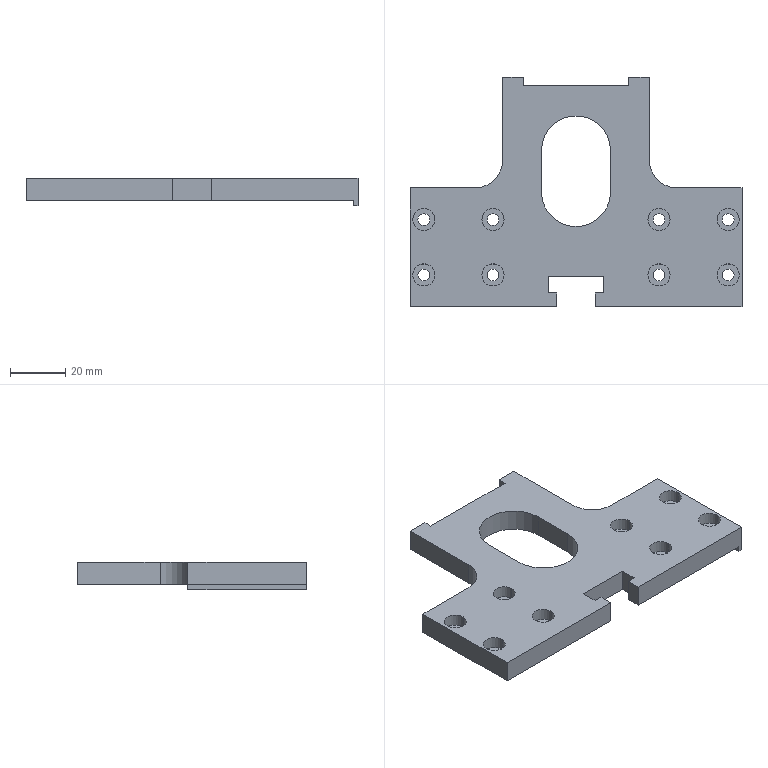Component | SolidWorks | HandlingMechanism-2_A069-1 | 1 solid | 78 faces | box 120 x 83 x 10 mm | volume 46963 mm3 | cylinder 40 | plane 34 | cone 4 | commonest cylinder face diameters 8 x16 4.3 x16 3.3 x4 25 x2 20 x2
build123d program:
from build123d import *

# Parameters (mm, degrees)
SKETCH1_W                                       = 120
SKETCH1_H                                       = 83
BOSS_EXTRUDE1_DEPTH                             = 10
SKETCH6_W                                       = 14
SKETCH6_H                                       = 5
CUT_EXTRUDE2_DEPTH                              = 15
SKETCH7_W                                       = 20
SKETCH7_H                                       = 6
CUT_EXTRUDE3_DEPTH                              = 15
SKETCH8_W                                       = 118.5
SKETCH8_H                                       = 83
CUT_EXTRUDE4_DEPTH                              = 2
SKETCH11_W                                      = 33.5
SKETCH11_H                                      = 40
CUT_EXTRUDE7_DEPTH                              = 20
SKETCH16_W                                      = 38
SKETCH16_H                                      = 3
CUT_EXTRUDE9_DEPTH                              = 20
M4_HEX_SOCKET_HEAD_CAP_SCREW_CBORE1_D           = 4.3
M4_HEX_SOCKET_HEAD_CAP_SCREW_CBORE1_CBORE_D     = 8
M4_HEX_SOCKET_HEAD_CAP_SCREW_CBORE1_CBORE_DEPTH = 4.4
CUT_EXTRUDE10_DEPTH                             = 74.636
M4_TAPPED_HOLE1_D                               = 3.3
M4_TAPPED_HOLE1_DEPTH                           = 11.5
M4_TAPPED_HOLE1_TIP                             = 0.9914
FILLET1_R                                       = 10


with BuildPart() as part:
    # Sketch1 → Boss-Extrude1 (new body)
    with BuildSketch(Plane.XY):
        Rectangle(SKETCH1_W, SKETCH1_H)
    extrude(amount=BOSS_EXTRUDE1_DEPTH)

    # Sketch6 → Cut-Extrude2 (cut)
    with BuildSketch(Plane.XY.offset(10)):
        with Locations((0, 39)):
            Rectangle(SKETCH6_W, SKETCH6_H)
    extrude(amount=-CUT_EXTRUDE2_DEPTH, mode=Mode.SUBTRACT)

    # Sketch7 → Cut-Extrude3 (cut)
    with BuildSketch(Plane.XY.offset(10)):
        with Locations((0, 33.5)):
            Rectangle(SKETCH7_W, SKETCH7_H)
    extrude(amount=-CUT_EXTRUDE3_DEPTH, mode=Mode.SUBTRACT)

    # Sketch8 → Cut-Extrude4 (cut)
    with BuildSketch(Plane(origin=(0, 0, 0), x_dir=(-1, 0, 0), z_dir=(0, 0, -1))):
        with Locations((-0.75, 0)):
            Rectangle(SKETCH8_W, SKETCH8_H)
    extrude(amount=-CUT_EXTRUDE4_DEPTH, mode=Mode.SUBTRACT)

    # Sketch11 → Cut-Extrude7 (cut)
    with BuildSketch(Plane.XY.offset(10)):
        with Locations((-43.25, -21.5)):
            Rectangle(SKETCH11_W, SKETCH11_H)
        with Locations((43.25, -21.5)):
            Rectangle(SKETCH11_W, SKETCH11_H)
    extrude(amount=-CUT_EXTRUDE7_DEPTH, mode=Mode.SUBTRACT)

    # Sketch16 → Cut-Extrude9 (cut)
    with BuildSketch(Plane(origin=(0, 0, 0), x_dir=(-1, 0, 0), z_dir=(0, 0, -1))):
        with Locations((0, -40)):
            Rectangle(SKETCH16_W, SKETCH16_H)
    extrude(amount=-CUT_EXTRUDE9_DEPTH, mode=Mode.SUBTRACT)

    # M4 Hex Socket Head Cap Screw CBORE1 (through all)
    with Locations(Plane.XY.offset(10)):
        with Locations((-55, 10), (-55, 30), (-30, 30), (-30, 10), (55, 30), (30, 30), (30, 10), (55, 10)):
            CounterBoreHole(M4_HEX_SOCKET_HEAD_CAP_SCREW_CBORE1_D / 2, M4_HEX_SOCKET_HEAD_CAP_SCREW_CBORE1_CBORE_D / 2, M4_HEX_SOCKET_HEAD_CAP_SCREW_CBORE1_CBORE_DEPTH)

    # Sketch19 → Cut-Extrude10 (cut, through all)
    with BuildSketch(Plane.XY.offset(10)):
        with BuildLine():
            Line((12.5, 0), (12.5, -15))
            ThreePointArc((12.5, -15), (0, -27.5), (-12.5, -15))
            Line((-12.5, -15), (-12.5, 0))
            ThreePointArc((-12.5, 0), (0, 12.5), (12.5, 0))
        make_face()
    extrude(amount=-CUT_EXTRUDE10_DEPTH, mode=Mode.SUBTRACT)

    # M4 Tapped Hole1
    with Locations(Plane(origin=(0, -38.5, 0), x_dir=(-1, 0, 0), z_dir=(0, -1, 0))):
        with Locations((14, -6), (-14, -6)):
            Hole(M4_TAPPED_HOLE1_D / 2, depth=M4_TAPPED_HOLE1_DEPTH)
            with Locations((0, 0, -(M4_TAPPED_HOLE1_DEPTH + M4_TAPPED_HOLE1_TIP / 2))):  # 118° drill point
                Cone(0, M4_TAPPED_HOLE1_D / 2, M4_TAPPED_HOLE1_TIP, mode=Mode.SUBTRACT)

    # Fillet1
    fillet1_edges = [part.edges().sort_by_distance(p)[0] for p in [
        (26.5, -1.5, 6),
        (-26.5, -1.5, 6),
    ]]
    fillet(fillet1_edges, radius=FILLET1_R)


solid = part.part

# Placed as in the assembly
solid = solid.moved(Location((25.881, 170, 147), (0, 0, 180)))